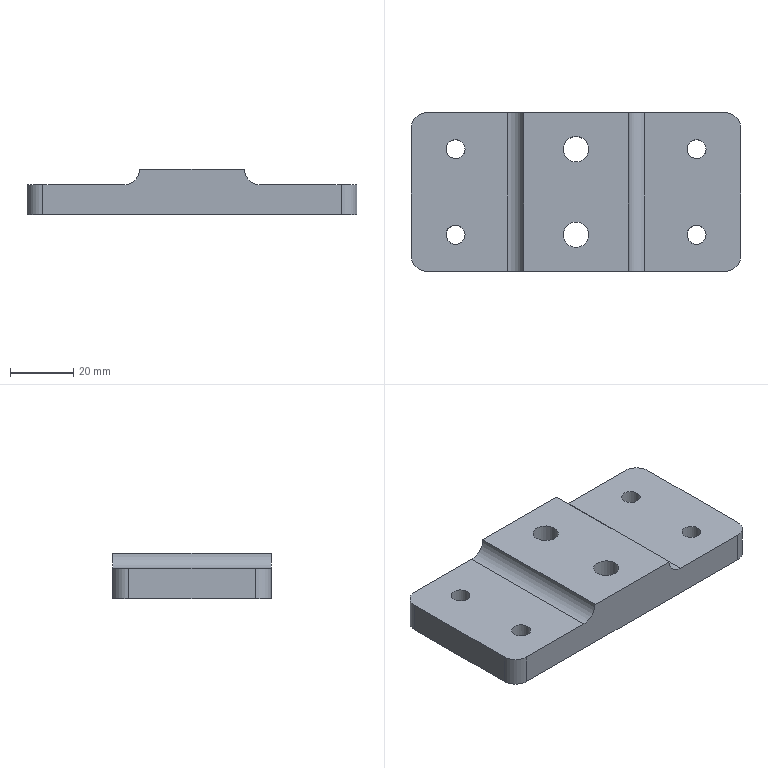Component | NX | CYLINDER_BODY_SUPPORT_LEG | 1 solid | 20 faces | volume 55451 mm3 | cylinder 12 | plane 8 | commonest cylinder face diameters 10 x6 6 x4 8 x2